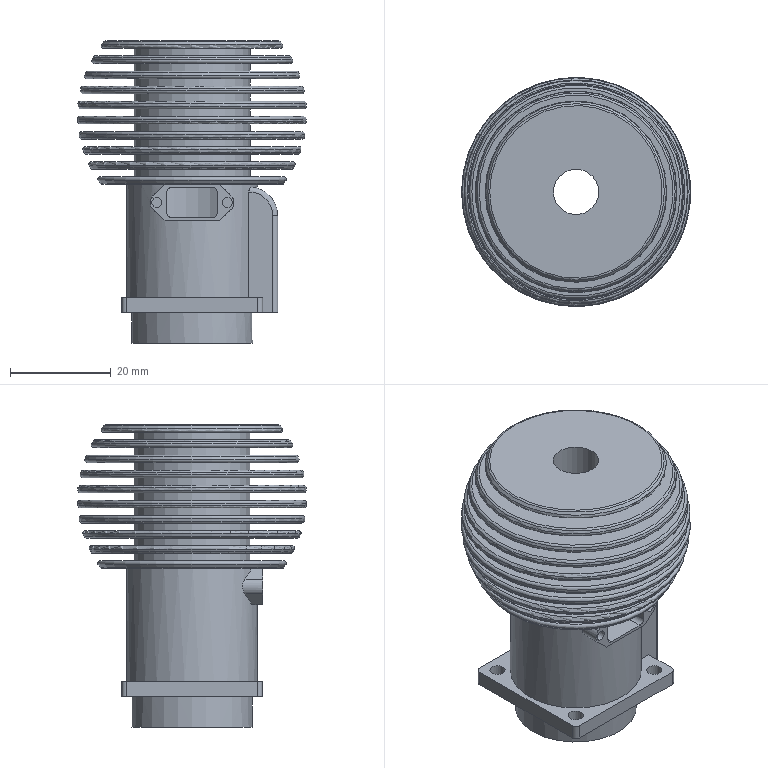Component | NX | PISTON_CYLINDER | 1 solid | 119 faces | volume 26453 mm3 | plane 53 | cylinder 34 | torus 22 | sphere 10 | commonest cylinder face diameters 2 x12 23 x9 3 x4 4 x2 20 x1 26 x1 24 x1 9 x1